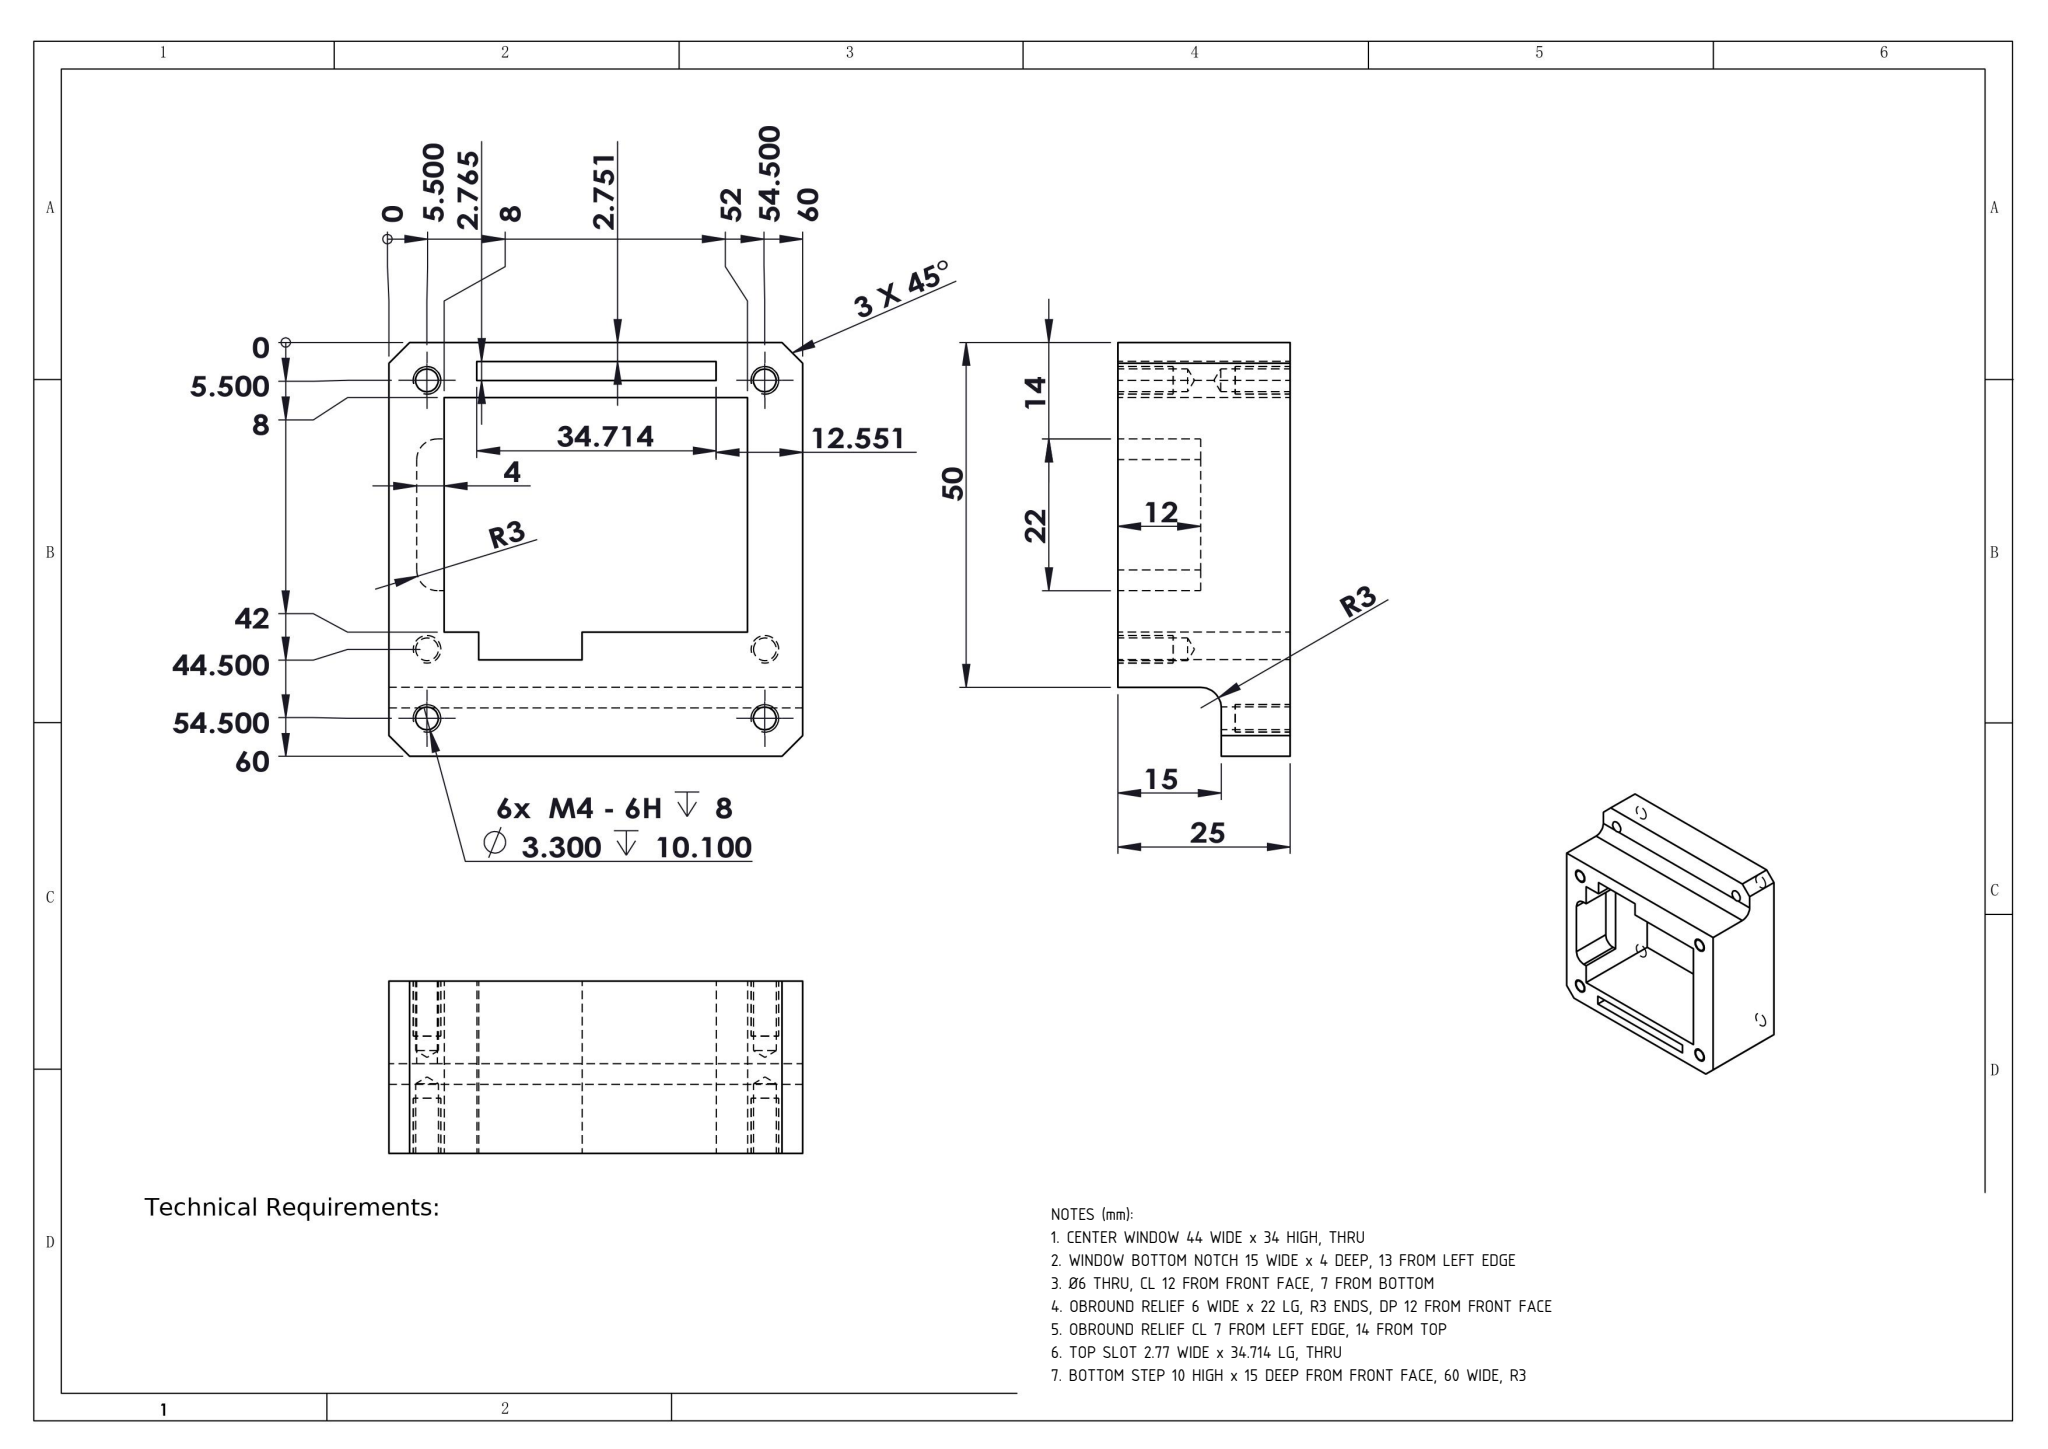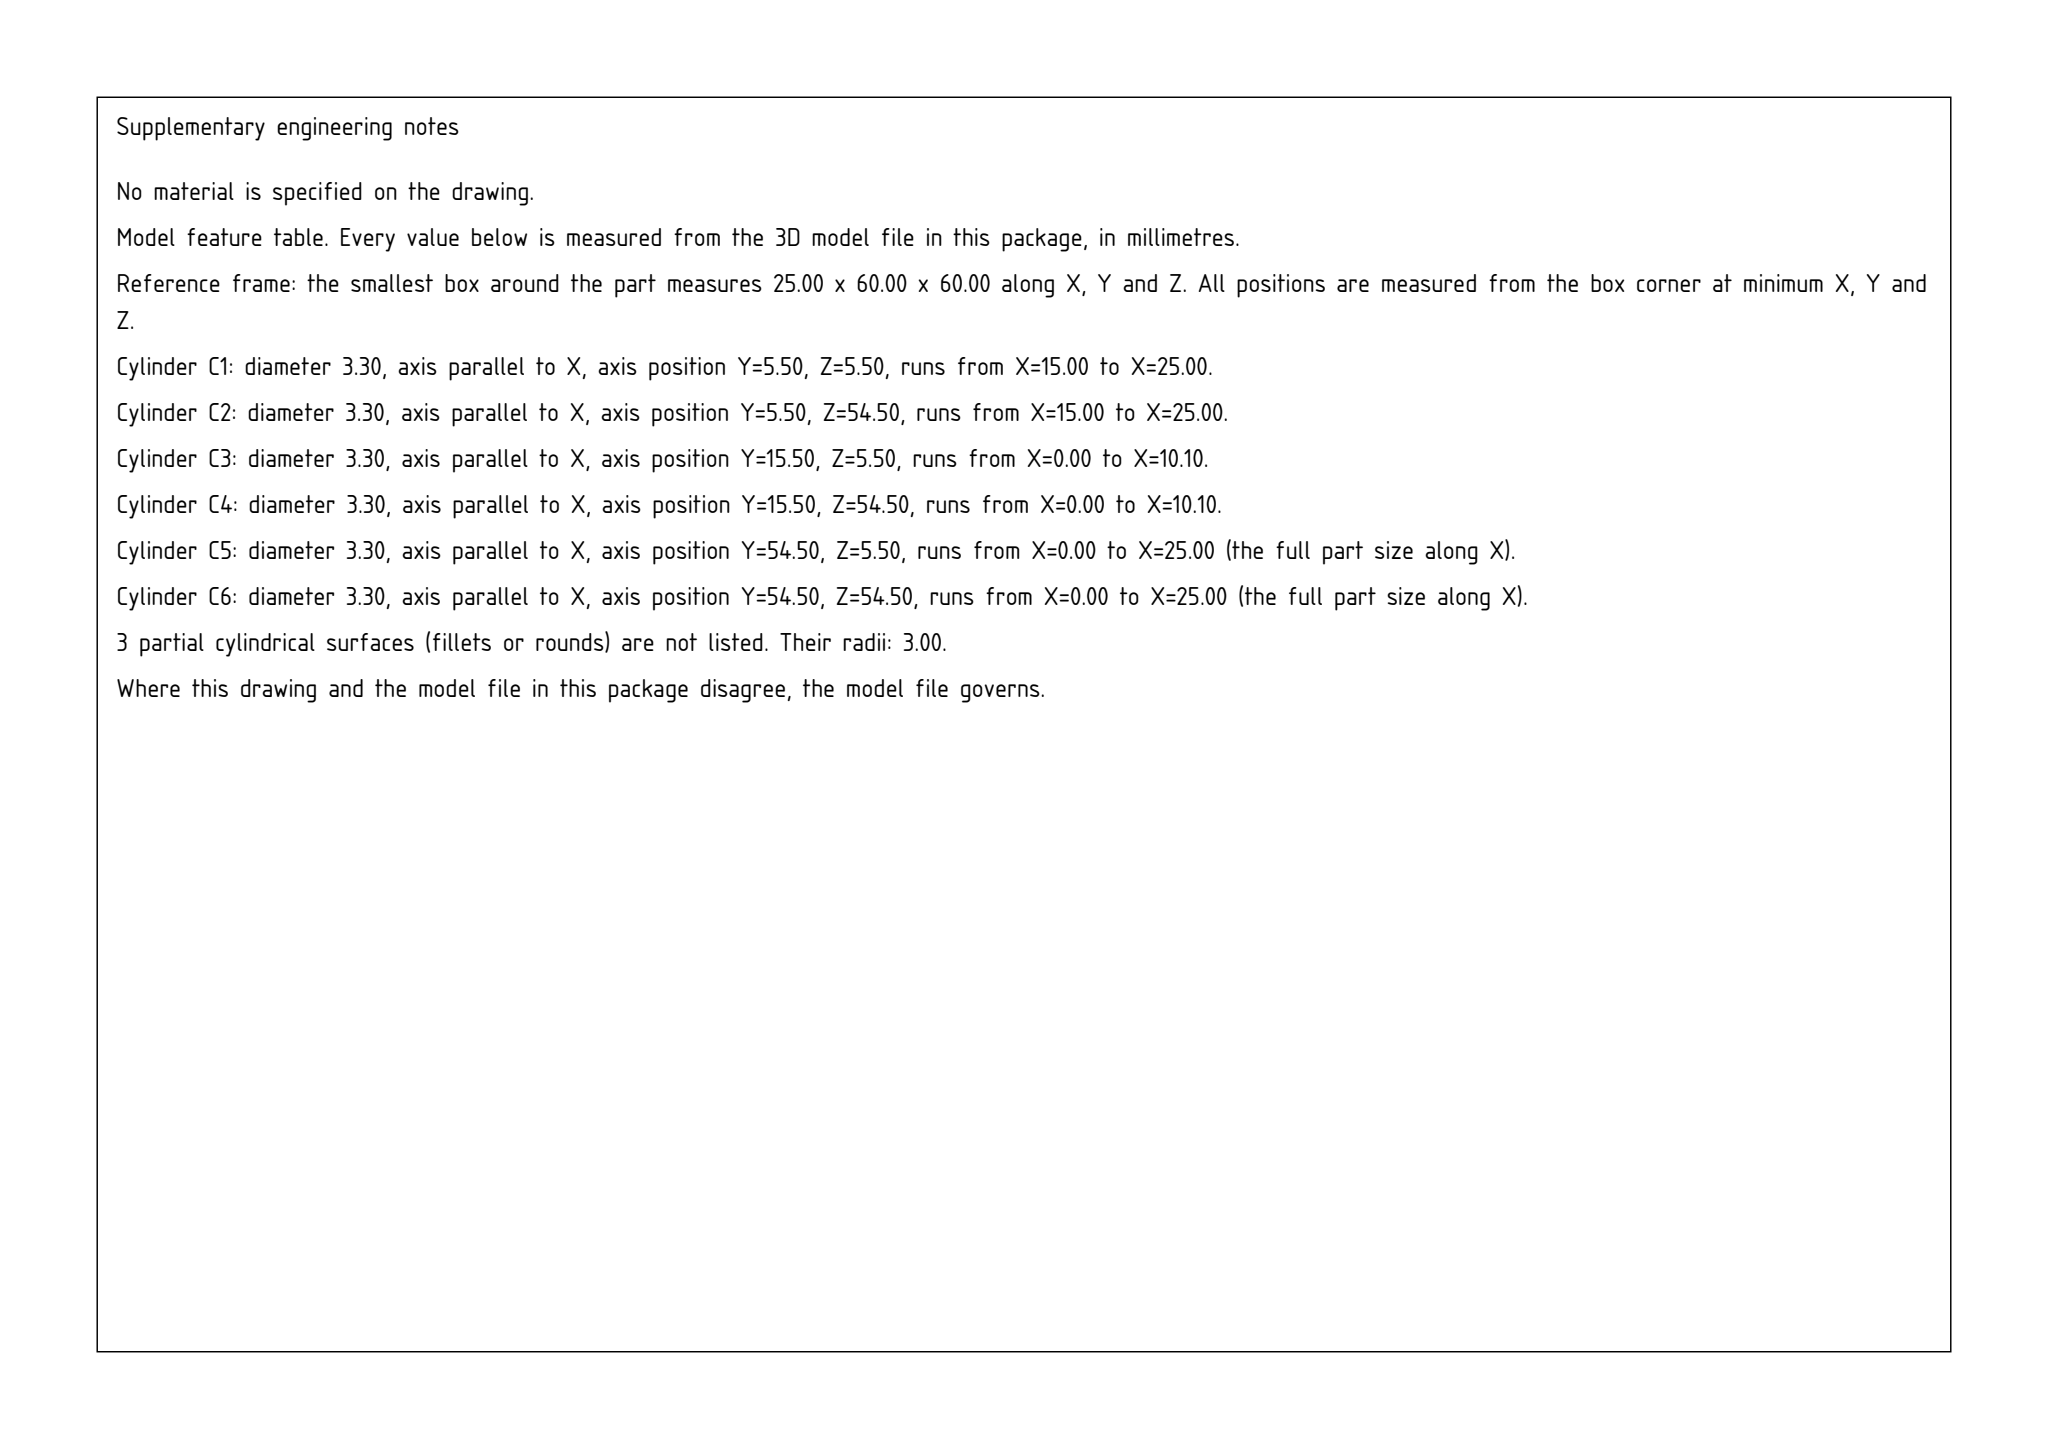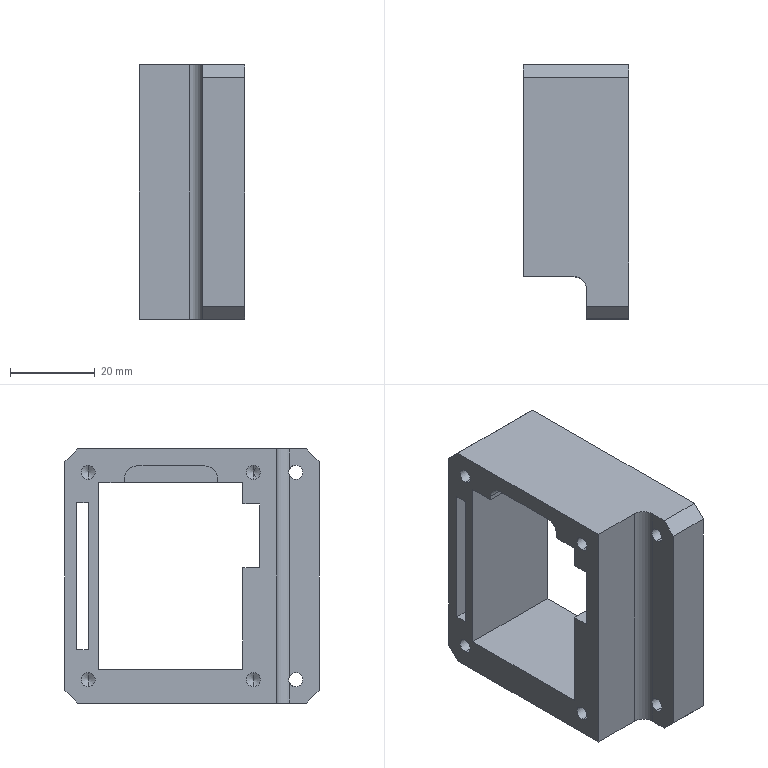Part | SolidWorks | mm | 1 solid | 59 faces | box 25 x 60 x 60 mm | volume 37785 mm3 | plane 28 | cylinder 19 | cone 12 | commonest cylinder face diameters 3.3 x16 6 x3
Drawing notes:
CENTER WINDOW 44 WIDE x 34 HIGH, THRU | from the solid: Window walls z=8 & 52 (44), y=18 & 52 (34); no X floor plane (x planes only 0,12,15,25) = thru
WINDOW BOTTOM NOTCH 15 WIDE x 4 DEEP, 13 FROM LEFT EDGE | from the solid: Notch walls z=32 & 47 (15 wide), floor y=14 vs window bottom y=18 (4 deep); 60-47=13 from drawing left edge
Ø6 THRU, CL 12 FROM FRONT FACE, 7 FROM BOTTOM | from the solid: cyl [6.0,'z',[12.0,7.0],60] - full 60 length = thru
OBROUND RELIEF 6 WIDE x 22 LG, R3 ENDS, DP 12 FROM FRONT FACE | from the solid: cyls [6.0,'x',[.,27,53],12] & [6.0,'x',[.,43,53],12]; y24-46=22 lg, 12 deep from x=0
OBROUND RELIEF CL 7 FROM LEFT EDGE, 14 FROM TOP | from the solid: z=53 -> 60-53=7 from drawing left edge; y=46 upper end -> 60-46=14 from top
TOP SLOT 2.77 WIDE x 34.714 LG, THRU | from the solid: y=54.48 & 57.25 (2.77 wide), z=12.55 & 47.26 (34.71 lg); no X floor plane = thru
BOTTOM STEP 10 HIGH x 15 DEEP FROM FRONT FACE, 60 WIDE, R3 | from the solid: y=0-10 step height, x=15 wall (25-15=10 remaining foot), full 60 in Z
build123d program:
from build123d import *

# Parameters (mm, degrees)
SKETCH1_W             = 60
SKETCH1_H             = 50
BOSS_EXTRUDE1_DEPTH   = 25
SKETCH2_W             = 10
SKETCH2_H             = 60
BOSS_EXTRUDE2_DEPTH   = 10
SKETCH5_W             = 44
SKETCH5_H             = 34
CUT_EXTRUDE1_DEPTH    = 49
CHAMFER1_SIZE         = 3
CUT_EXTRUDE2_DEPTH    = 12
FILLET3_R             = 3
M4_TAPPED_HOLE1_D     = 3.3
M4_TAPPED_HOLE1_DEPTH = 10.1
M4_TAPPED_HOLE1_TIP   = 0.9914
M4_TAPPED_HOLE2_D     = 3.3
M4_TAPPED_HOLE2_DEPTH = 10.1
M4_TAPPED_HOLE2_TIP   = 0.9914
SKETCH12_W            = 15
SKETCH12_H            = 13.918
CUT_EXTRUDE4_DEPTH    = 83.006
SKETCH13_W            = 34.714
SKETCH13_H            = 2.765
CUT_EXTRUDE5_DEPTH    = 49


with BuildPart() as part:
    # Sketch1 → Boss-Extrude1 (new body)
    with BuildSketch(Plane(origin=(0, 0, 0), x_dir=(0, 0, -1), z_dir=(1, 0, 0))):
        with Locations((30, 25)):
            Rectangle(SKETCH1_W, SKETCH1_H)
    extrude(amount=BOSS_EXTRUDE1_DEPTH)

    # Sketch2 → Boss-Extrude2 (add)
    with BuildSketch(Plane.XZ):
        with Locations((20, -30)):
            Rectangle(SKETCH2_W, SKETCH2_H)
    extrude(amount=BOSS_EXTRUDE2_DEPTH)

    # Sketch5 → Cut-Extrude1 (cut)
    with BuildSketch(Plane(origin=(25, 0, 0), x_dir=(0, 0, -1), z_dir=(1, 0, 0))):
        with Locations((30, 25)):
            Rectangle(SKETCH5_W, SKETCH5_H)
    extrude(amount=-CUT_EXTRUDE1_DEPTH, mode=Mode.SUBTRACT)

    # Chamfer1
    chamfer1_edges = [part.edges().sort_by_distance(p)[0] for p in [
        (12.5, 50, -60),
        (12.5, 50, 0),
        (20, -10, -60),
        (20, -10, 0),
    ]]
    chamfer(chamfer1_edges, length=CHAMFER1_SIZE)

    # Sketch6 → Cut-Extrude2 (cut)
    with BuildSketch(Plane.ZY):
        with BuildLine():
            Line((-8, 14), (-7, 14))
            ThreePointArc((-7, 14), (-4.879, 14.879), (-4, 17))
            Line((-4, 17), (-4, 33))
            ThreePointArc((-4, 33), (-4.879, 35.121), (-7, 36))
            Line((-7, 36), (-8, 36))
            Line((-8, 36), (-8, 14))
        make_face()
    extrude(amount=-CUT_EXTRUDE2_DEPTH, mode=Mode.SUBTRACT)

    # Fillet3
    fillet3_edges = [part.edges().sort_by_distance(p)[0] for p in [
        (15, 0, -30),
    ]]
    fillet(fillet3_edges, radius=FILLET3_R)

    # M4 Tapped Hole1
    with Locations(Plane(origin=(25, 0, 0), x_dir=(0, 0, -1), z_dir=(1, 0, 0))):
        with Locations((54.5, -4.5), (5.5, -4.5), (54.5, 44.5), (5.5, 44.5)):
            Hole(M4_TAPPED_HOLE1_D / 2, depth=M4_TAPPED_HOLE1_DEPTH)
            with Locations((0, 0, -(M4_TAPPED_HOLE1_DEPTH + M4_TAPPED_HOLE1_TIP / 2))):  # 118° drill point
                Cone(0, M4_TAPPED_HOLE1_D / 2, M4_TAPPED_HOLE1_TIP, mode=Mode.SUBTRACT)

    # M4 Tapped Hole2
    with Locations(Plane.ZY):
        with Locations((-5.5, 44.5), (-54.5, 44.5), (-54.5, 5.5), (-5.5, 5.5)):
            Hole(M4_TAPPED_HOLE2_D / 2, depth=M4_TAPPED_HOLE2_DEPTH)
            with Locations((0, 0, -(M4_TAPPED_HOLE2_DEPTH + M4_TAPPED_HOLE2_TIP / 2))):  # 118° drill point
                Cone(0, M4_TAPPED_HOLE2_D / 2, M4_TAPPED_HOLE2_TIP, mode=Mode.SUBTRACT)

    # Sketch12 → Cut-Extrude4 (cut, through all)
    with BuildSketch(Plane(origin=(25, 0, 0), x_dir=(0, 0, -1), z_dir=(1, 0, 0))):
        with Locations((20.5, 10.959)):
            Rectangle(SKETCH12_W, SKETCH12_H)
    extrude(amount=-CUT_EXTRUDE4_DEPTH, mode=Mode.SUBTRACT)

    # Sketch13 → Cut-Extrude5 (cut)
    with BuildSketch(Plane.ZY):
        with Locations((-30.092, 45.866)):
            Rectangle(SKETCH13_W, SKETCH13_H)
    extrude(amount=-CUT_EXTRUDE5_DEPTH, mode=Mode.SUBTRACT)


solid = part.part